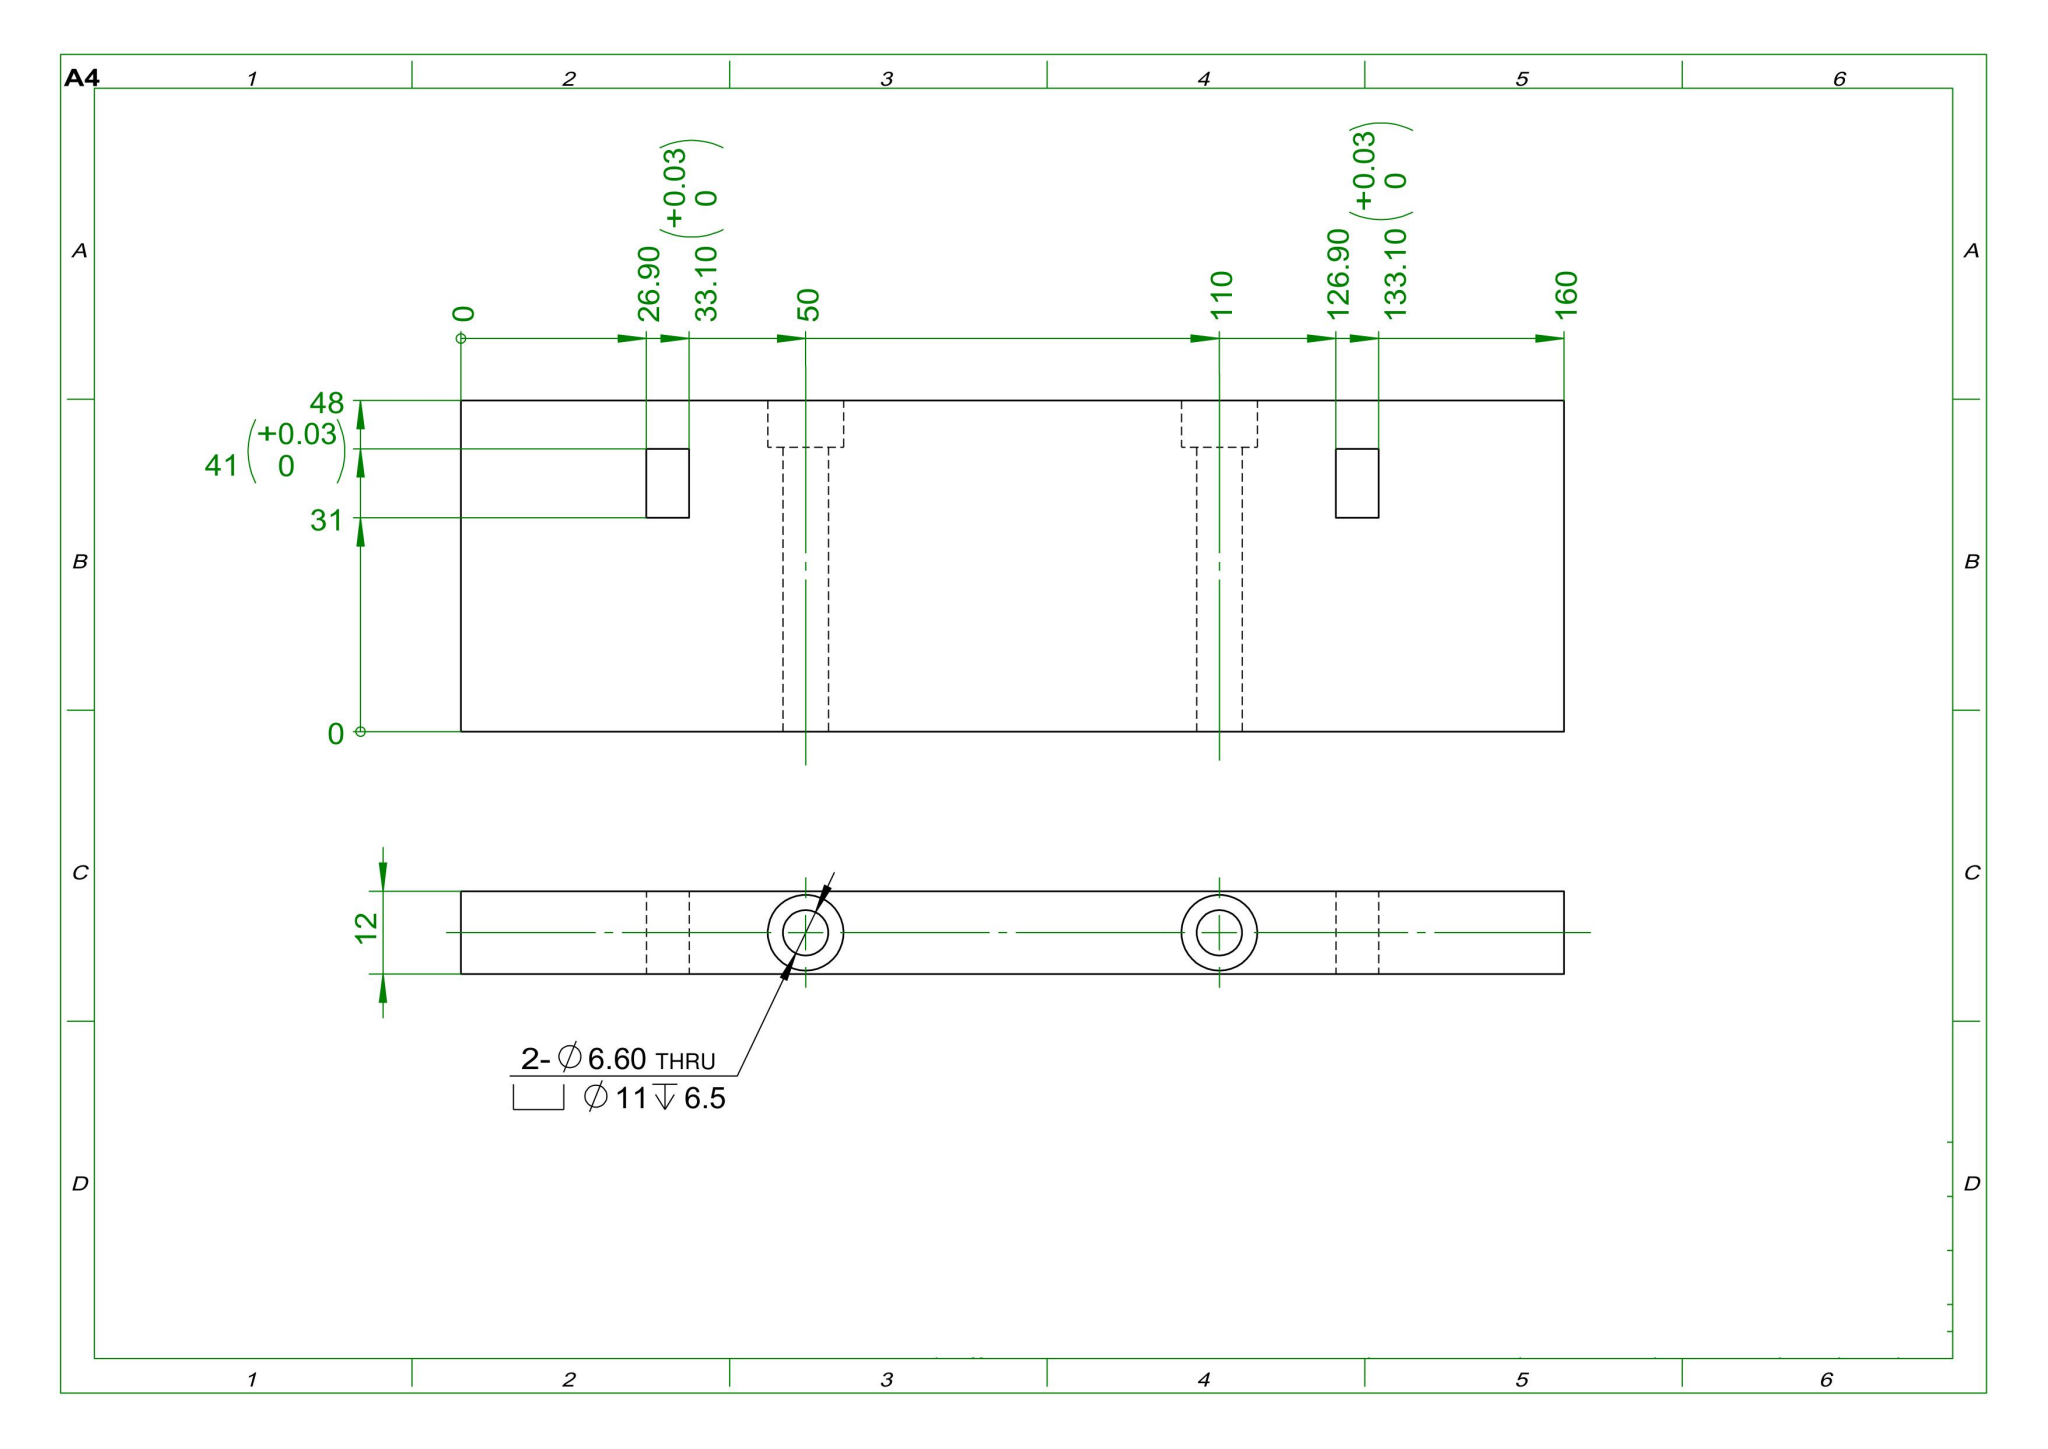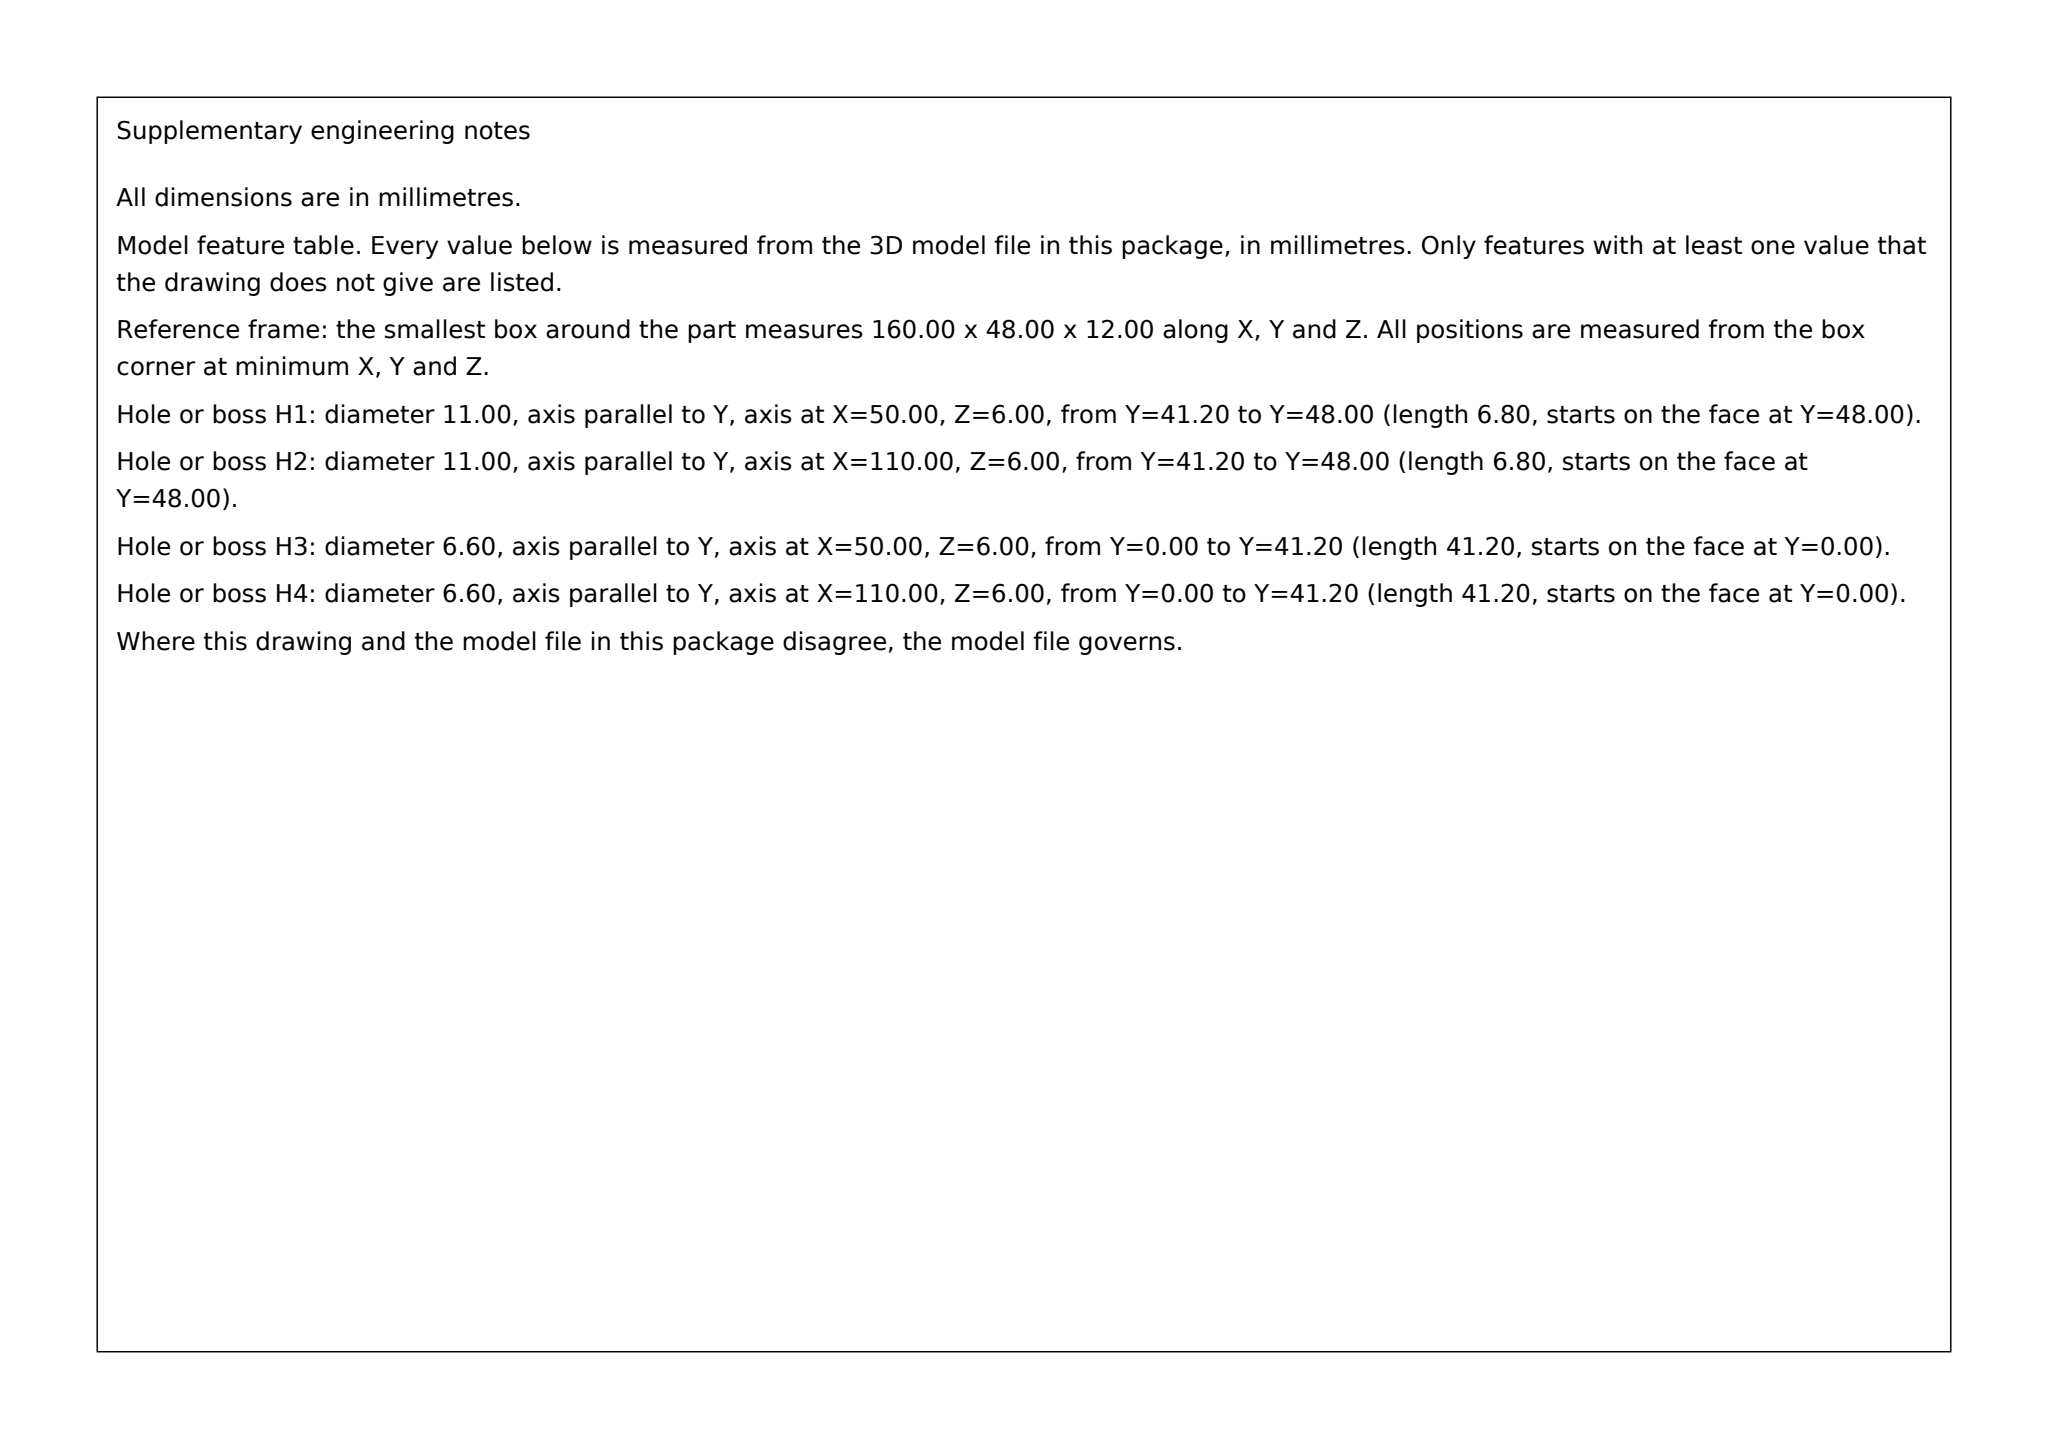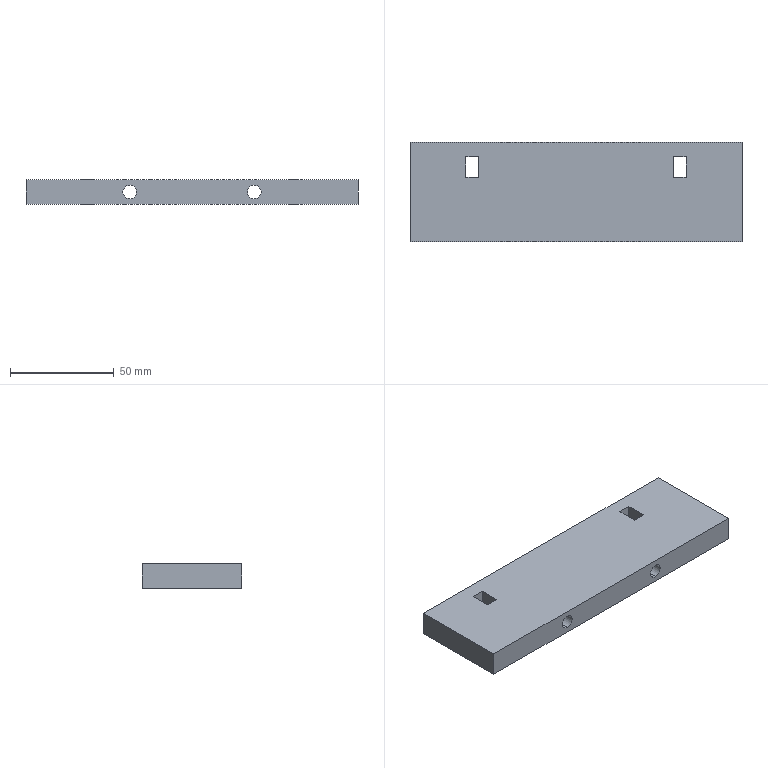Part | SolidWorks | mm | 1 solid | 24 faces | box 160 x 48 x 12 mm | volume 86560 mm3 | plane 16 | cylinder 8 | commonest cylinder face diameters 11 x4 6.6 x4
build123d program:
from build123d import *

# Parameters (mm, degrees)
SKETCH1_W                                            = 160
SKETCH1_H                                            = 48
SKETCH1_W_2                                          = 6.2
SKETCH1_H_2                                          = 10
BOSS_EXTRUDE1_DEPTH                                  = 12
HOLE_SIZE_ACCORDING_TO_HEXAGON_SOCKET_HE_D           = 6.6
HOLE_SIZE_ACCORDING_TO_HEXAGON_SOCKET_HE_CBORE_D     = 11
HOLE_SIZE_ACCORDING_TO_HEXAGON_SOCKET_HE_CBORE_DEPTH = 6.8


with BuildPart() as part:
    # Sketch1 → Boss-Extrude1 (new body)
    with BuildSketch(Plane.XY):
        Rectangle(SKETCH1_W, SKETCH1_H)
        with Locations((50, 12)):
            Rectangle(SKETCH1_W_2, SKETCH1_H_2, mode=Mode.SUBTRACT)
        with Locations((-50, 12)):
            Rectangle(SKETCH1_W_2, SKETCH1_H_2, mode=Mode.SUBTRACT)
    extrude(amount=BOSS_EXTRUDE1_DEPTH)

    # Hole Size_according to_Hexagon Socket He (through all)
    with Locations(Plane(origin=(0, 24, 0), x_dir=(1, 0, 0), z_dir=(0, 1, 0))):
        with Locations((-30, -6), (30, -6)):
            CounterBoreHole(HOLE_SIZE_ACCORDING_TO_HEXAGON_SOCKET_HE_D / 2, HOLE_SIZE_ACCORDING_TO_HEXAGON_SOCKET_HE_CBORE_D / 2, HOLE_SIZE_ACCORDING_TO_HEXAGON_SOCKET_HE_CBORE_DEPTH)


solid = part.part
STEP:
#1=CARTESIAN_POINT('',(-30.,17.2,0.5));
#2=VERTEX_POINT('',#1);
#3=CARTESIAN_POINT('',(-30.,17.2,11.5));
#4=VERTEX_POINT('',#3);
#5=CARTESIAN_POINT('',(-30.,17.2,6.));
#6=DIRECTION('',(0.,1.,0.));
#7=DIRECTION('',(0.,0.,1.));
#8=AXIS2_PLACEMENT_3D('',#5,#6,#7);
#9=CIRCLE('',#8,5.5);
#10=EDGE_CURVE('',#2,#4,#9,.T.);
#11=ORIENTED_EDGE('',*,*,#10,.F.);
#12=CARTESIAN_POINT('',(-30.,24.,0.5));
#13=VERTEX_POINT('',#12);
#14=CARTESIAN_POINT('',(-30.,24.,0.5));
#15=DIRECTION('',(0.,1.,0.));
#16=VECTOR('',#15,1000.);
#17=LINE('',#14,#16);
#18=EDGE_CURVE('',#2,#13,#17,.T.);
#19=ORIENTED_EDGE('',*,*,#18,.T.);
#20=CARTESIAN_POINT('',(-30.,24.,11.5));
#21=VERTEX_POINT('',#20);
#22=CARTESIAN_POINT('',(-30.,24.,6.));
#23=DIRECTION('',(0.,1.,0.));
#24=DIRECTION('',(0.,0.,1.));
#25=AXIS2_PLACEMENT_3D('',#22,#23,#24);
#26=CIRCLE('',#25,5.5);
#27=EDGE_CURVE('',#13,#21,#26,.T.);
#28=ORIENTED_EDGE('',*,*,#27,.T.);
#29=CARTESIAN_POINT('',(-30.,24.,11.5));
#30=DIRECTION('',(0.,1.,0.));
#31=VECTOR('',#30,1000.);
#32=LINE('',#29,#31);
#33=EDGE_CURVE('',#4,#21,#32,.T.);
#34=ORIENTED_EDGE('',*,*,#33,.F.);
#35=EDGE_LOOP('',(#11,#19,#28,#34));
#36=FACE_OUTER_BOUND('',#35,.T.);
#37=CARTESIAN_POINT('',(-30.,24.,6.));
#38=DIRECTION('',(0.,1.,0.));
#39=DIRECTION('',(0.,0.,1.));
#40=AXIS2_PLACEMENT_3D('',#37,#38,#39);
#41=CYLINDRICAL_SURFACE('',#40,5.5);
#42=ADVANCED_FACE('',(#36),#41,.F.);
#43=CARTESIAN_POINT('',(-30.,-24.,2.7));
#44=VERTEX_POINT('',#43);
#45=CARTESIAN_POINT('',(-30.,-24.,9.3));
#46=VERTEX_POINT('',#45);
#47=CARTESIAN_POINT('',(-30.,-24.,6.));
#48=DIRECTION('',(0.,1.,0.));
#49=DIRECTION('',(0.,0.,1.));
#50=AXIS2_PLACEMENT_3D('',#47,#48,#49);
#51=CIRCLE('',#50,3.3);
#52=EDGE_CURVE('',#44,#46,#51,.T.);
#53=ORIENTED_EDGE('',*,*,#52,.F.);
#54=CARTESIAN_POINT('',(-30.,17.2,2.7));
#55=VERTEX_POINT('',#54);
#56=CARTESIAN_POINT('',(-30.,24.,2.7));
#57=DIRECTION('',(0.,1.,0.));
#58=VECTOR('',#57,1000.);
#59=LINE('',#56,#58);
#60=EDGE_CURVE('',#44,#55,#59,.T.);
#61=ORIENTED_EDGE('',*,*,#60,.T.);
#62=CARTESIAN_POINT('',(-30.,17.2,9.3));
#63=VERTEX_POINT('',#62);
#64=CARTESIAN_POINT('',(-30.,17.2,6.));
#65=DIRECTION('',(0.,1.,0.));
#66=DIRECTION('',(0.,0.,1.));
#67=AXIS2_PLACEMENT_3D('',#64,#65,#66);
#68=CIRCLE('',#67,3.3);
#69=EDGE_CURVE('',#55,#63,#68,.T.);
#70=ORIENTED_EDGE('',*,*,#69,.T.);
#71=CARTESIAN_POINT('',(-30.,24.,9.3));
#72=DIRECTION('',(0.,1.,0.));
#73=VECTOR('',#72,1000.);
#74=LINE('',#71,#73);
#75=EDGE_CURVE('',#46,#63,#74,.T.);
#76=ORIENTED_EDGE('',*,*,#75,.F.);
#77=EDGE_LOOP('',(#53,#61,#70,#76));
#78=FACE_OUTER_BOUND('',#77,.T.);
#79=CARTESIAN_POINT('',(-30.,24.,6.));
#80=DIRECTION('',(0.,1.,0.));
#81=DIRECTION('',(0.,0.,1.));
#82=AXIS2_PLACEMENT_3D('',#79,#80,#81);
#83=CYLINDRICAL_SURFACE('',#82,3.3);
#84=ADVANCED_FACE('',(#78),#83,.F.);
#85=CARTESIAN_POINT('',(30.,17.2,0.5));
#86=VERTEX_POINT('',#85);
#87=CARTESIAN_POINT('',(30.,17.2,11.5));
#88=VERTEX_POINT('',#87);
#89=CARTESIAN_POINT('',(30.,17.2,6.));
#90=DIRECTION('',(0.,1.,0.));
#91=DIRECTION('',(0.,0.,1.));
#92=AXIS2_PLACEMENT_3D('',#89,#90,#91);
#93=CIRCLE('',#92,5.5);
#94=EDGE_CURVE('',#86,#88,#93,.T.);
#95=ORIENTED_EDGE('',*,*,#94,.F.);
#96=CARTESIAN_POINT('',(30.,24.,0.5));
#97=VERTEX_POINT('',#96);
#98=CARTESIAN_POINT('',(30.,24.,0.5));
#99=DIRECTION('',(0.,1.,0.));
#100=VECTOR('',#99,1000.);
#101=LINE('',#98,#100);
#102=EDGE_CURVE('',#86,#97,#101,.T.);
#103=ORIENTED_EDGE('',*,*,#102,.T.);
#104=CARTESIAN_POINT('',(30.,24.,11.5));
#105=VERTEX_POINT('',#104);
#106=CARTESIAN_POINT('',(30.,24.,6.));
#107=DIRECTION('',(0.,1.,0.));
#108=DIRECTION('',(0.,0.,1.));
#109=AXIS2_PLACEMENT_3D('',#106,#107,#108);
#110=CIRCLE('',#109,5.5);
#111=EDGE_CURVE('',#97,#105,#110,.T.);
#112=ORIENTED_EDGE('',*,*,#111,.T.);
#113=CARTESIAN_POINT('',(30.,24.,11.5));
#114=DIRECTION('',(0.,1.,0.));
#115=VECTOR('',#114,1000.);
#116=LINE('',#113,#115);
#117=EDGE_CURVE('',#88,#105,#116,.T.);
#118=ORIENTED_EDGE('',*,*,#117,.F.);
#119=EDGE_LOOP('',(#95,#103,#112,#118));
#120=FACE_OUTER_BOUND('',#119,.T.);
#121=CARTESIAN_POINT('',(30.,24.,6.));
#122=DIRECTION('',(0.,1.,0.));
#123=DIRECTION('',(0.,0.,1.));
#124=AXIS2_PLACEMENT_3D('',#121,#122,#123);
#125=CYLINDRICAL_SURFACE('',#124,5.5);
#126=ADVANCED_FACE('',(#120),#125,.F.);
#127=CARTESIAN_POINT('',(30.,-24.,2.7));
#128=VERTEX_POINT('',#127);
#129=CARTESIAN_POINT('',(30.,-24.,9.3));
#130=VERTEX_POINT('',#129);
#131=CARTESIAN_POINT('',(30.,-24.,6.));
#132=DIRECTION('',(0.,1.,0.));
#133=DIRECTION('',(0.,0.,1.));
#134=AXIS2_PLACEMENT_3D('',#131,#132,#133);
#135=CIRCLE('',#134,3.3);
#136=EDGE_CURVE('',#128,#130,#135,.T.);
#137=ORIENTED_EDGE('',*,*,#136,.F.);
#138=CARTESIAN_POINT('',(30.,17.2,2.7));
#139=VERTEX_POINT('',#138);
#140=CARTESIAN_POINT('',(30.,24.,2.7));
#141=DIRECTION('',(0.,1.,0.));
#142=VECTOR('',#141,1000.);
#143=LINE('',#140,#142);
#144=EDGE_CURVE('',#128,#139,#143,.T.);
#145=ORIENTED_EDGE('',*,*,#144,.T.);
#146=CARTESIAN_POINT('',(30.,17.2,9.3));
#147=VERTEX_POINT('',#146);
#148=CARTESIAN_POINT('',(30.,17.2,6.));
#149=DIRECTION('',(0.,1.,0.));
#150=DIRECTION('',(0.,0.,1.));
#151=AXIS2_PLACEMENT_3D('',#148,#149,#150);
#152=CIRCLE('',#151,3.3);
#153=EDGE_CURVE('',#139,#147,#152,.T.);
#154=ORIENTED_EDGE('',*,*,#153,.T.);
#155=CARTESIAN_POINT('',(30.,24.,9.3));
#156=DIRECTION('',(0.,1.,0.));
#157=VECTOR('',#156,1000.);
#158=LINE('',#155,#157);
#159=EDGE_CURVE('',#130,#147,#158,.T.);
#160=ORIENTED_EDGE('',*,*,#159,.F.);
#161=EDGE_LOOP('',(#137,#145,#154,#160));
#162=FACE_OUTER_BOUND('',#161,.T.);
#163=CARTESIAN_POINT('',(30.,24.,6.));
#164=DIRECTION('',(0.,1.,0.));
#165=DIRECTION('',(0.,0.,1.));
#166=AXIS2_PLACEMENT_3D('',#163,#164,#165);
#167=CYLINDRICAL_SURFACE('',#166,3.3);
#168=ADVANCED_FACE('',(#162),#167,.F.);
#169=CARTESIAN_POINT('',(-46.9,7.,12.));
#170=VERTEX_POINT('',#169);
#171=CARTESIAN_POINT('',(-46.9,17.,12.));
#172=VERTEX_POINT('',#171);
#173=CARTESIAN_POINT('',(-46.9,7.,12.));
#174=DIRECTION('',(0.,1.,0.));
#175=VECTOR('',#174,1000.);
#176=LINE('',#173,#175);
#177=EDGE_CURVE('',#170,#172,#176,.T.);
#178=ORIENTED_EDGE('',*,*,#177,.F.);
#179=CARTESIAN_POINT('',(-53.1,7.,12.));
#180=VERTEX_POINT('',#179);
#181=CARTESIAN_POINT('',(-53.1,7.,12.));
#182=DIRECTION('',(1.,0.,0.));
#183=VECTOR('',#182,1000.);
#184=LINE('',#181,#183);
#185=EDGE_CURVE('',#180,#170,#184,.T.);
#186=ORIENTED_EDGE('',*,*,#185,.F.);
#187=CARTESIAN_POINT('',(-53.1,17.,12.));
#188=VERTEX_POINT('',#187);
#189=CARTESIAN_POINT('',(-53.1,7.,12.));
#190=DIRECTION('',(0.,-1.,0.));
#191=VECTOR('',#190,1000.);
#192=LINE('',#189,#191);
#193=EDGE_CURVE('',#188,#180,#192,.T.);
#194=ORIENTED_EDGE('',*,*,#193,.F.);
#195=CARTESIAN_POINT('',(-53.1,17.,12.));
#196=DIRECTION('',(-1.,0.,0.));
#197=VECTOR('',#196,1000.);
#198=LINE('',#195,#197);
#199=EDGE_CURVE('',#172,#188,#198,.T.);
#200=ORIENTED_EDGE('',*,*,#199,.F.);
#201=EDGE_LOOP('',(#178,#186,#194,#200));
#202=FACE_BOUND('',#201,.T.);
#203=CARTESIAN_POINT('',(80.,-24.,12.));
#204=VERTEX_POINT('',#203);
#205=CARTESIAN_POINT('',(80.,24.,12.));
#206=VERTEX_POINT('',#205);
#207=CARTESIAN_POINT('',(80.,-24.,12.));
#208=DIRECTION('',(0.,1.,0.));
#209=VECTOR('',#208,1000.);
#210=LINE('',#207,#209);
#211=EDGE_CURVE('',#204,#206,#210,.T.);
#212=ORIENTED_EDGE('',*,*,#211,.T.);
#213=CARTESIAN_POINT('',(-80.,24.,12.));
#214=VERTEX_POINT('',#213);
#215=CARTESIAN_POINT('',(-80.,24.,12.));
#216=DIRECTION('',(-1.,0.,0.));
#217=VECTOR('',#216,1000.);
#218=LINE('',#215,#217);
#219=EDGE_CURVE('',#206,#214,#218,.T.);
#220=ORIENTED_EDGE('',*,*,#219,.T.);
#221=CARTESIAN_POINT('',(-80.,-24.,12.));
#222=VERTEX_POINT('',#221);
#223=CARTESIAN_POINT('',(-80.,-24.,12.));
#224=DIRECTION('',(0.,-1.,0.));
#225=VECTOR('',#224,1000.);
#226=LINE('',#223,#225);
#227=EDGE_CURVE('',#214,#222,#226,.T.);
#228=ORIENTED_EDGE('',*,*,#227,.T.);
#229=CARTESIAN_POINT('',(-80.,-24.,12.));
#230=DIRECTION('',(1.,0.,0.));
#231=VECTOR('',#230,1000.);
#232=LINE('',#229,#231);
#233=EDGE_CURVE('',#222,#204,#232,.T.);
#234=ORIENTED_EDGE('',*,*,#233,.T.);
#235=EDGE_LOOP('',(#212,#220,#228,#234));
#236=FACE_OUTER_BOUND('',#235,.T.);
#237=CARTESIAN_POINT('',(53.1,7.,12.));
#238=VERTEX_POINT('',#237);
#239=CARTESIAN_POINT('',(53.1,17.,12.));
#240=VERTEX_POINT('',#239);
#241=CARTESIAN_POINT('',(53.1,7.,12.));
#242=DIRECTION('',(0.,1.,0.));
#243=VECTOR('',#242,1000.);
#244=LINE('',#241,#243);
#245=EDGE_CURVE('',#238,#240,#244,.T.);
#246=ORIENTED_EDGE('',*,*,#245,.F.);
#247=CARTESIAN_POINT('',(46.9,7.,12.));
#248=VERTEX_POINT('',#247);
#249=CARTESIAN_POINT('',(53.1,7.,12.));
#250=DIRECTION('',(1.,0.,0.));
#251=VECTOR('',#250,1000.);
#252=LINE('',#249,#251);
#253=EDGE_CURVE('',#248,#238,#252,.T.);
#254=ORIENTED_EDGE('',*,*,#253,.F.);
#255=CARTESIAN_POINT('',(46.9,17.,12.));
#256=VERTEX_POINT('',#255);
#257=CARTESIAN_POINT('',(46.9,7.,12.));
#258=DIRECTION('',(0.,-1.,0.));
#259=VECTOR('',#258,1000.);
#260=LINE('',#257,#259);
#261=EDGE_CURVE('',#256,#248,#260,.T.);
#262=ORIENTED_EDGE('',*,*,#261,.F.);
#263=CARTESIAN_POINT('',(53.1,17.,12.));
#264=DIRECTION('',(-1.,0.,0.));
#265=VECTOR('',#264,1000.);
#266=LINE('',#263,#265);
#267=EDGE_CURVE('',#240,#256,#266,.T.);
#268=ORIENTED_EDGE('',*,*,#267,.F.);
#269=EDGE_LOOP('',(#246,#254,#262,#268));
#270=FACE_BOUND('',#269,.T.);
#271=CARTESIAN_POINT('',(0.,0.,12.));
#272=DIRECTION('',(0.,0.,-1.));
#273=DIRECTION('',(-1.,0.,0.));
#274=AXIS2_PLACEMENT_3D('',#271,#272,#273);
#275=PLANE('',#274);
#276=ADVANCED_FACE('',(#202,#236,#270),#275,.F.);
#277=CARTESIAN_POINT('',(-53.1,7.,0.));
#278=VERTEX_POINT('',#277);
#279=CARTESIAN_POINT('',(-46.9,7.,0.));
#280=VERTEX_POINT('',#279);
#281=CARTESIAN_POINT('',(-53.1,7.,0.));
#282=DIRECTION('',(1.,0.,0.));
#283=VECTOR('',#282,1000.);
#284=LINE('',#281,#283);
#285=EDGE_CURVE('',#278,#280,#284,.T.);
#286=ORIENTED_EDGE('',*,*,#285,.T.);
#287=CARTESIAN_POINT('',(-46.9,17.,0.));
#288=VERTEX_POINT('',#287);
#289=CARTESIAN_POINT('',(-46.9,7.,0.));
#290=DIRECTION('',(0.,1.,0.));
#291=VECTOR('',#290,1000.);
#292=LINE('',#289,#291);
#293=EDGE_CURVE('',#280,#288,#292,.T.);
#294=ORIENTED_EDGE('',*,*,#293,.T.);
#295=CARTESIAN_POINT('',(-53.1,17.,0.));
#296=VERTEX_POINT('',#295);
#297=CARTESIAN_POINT('',(-53.1,17.,0.));
#298=DIRECTION('',(-1.,0.,0.));
#299=VECTOR('',#298,1000.);
#300=LINE('',#297,#299);
#301=EDGE_CURVE('',#288,#296,#300,.T.);
#302=ORIENTED_EDGE('',*,*,#301,.T.);
#303=CARTESIAN_POINT('',(-53.1,7.,0.));
#304=DIRECTION('',(0.,-1.,0.));
#305=VECTOR('',#304,1000.);
#306=LINE('',#303,#305);
#307=EDGE_CURVE('',#296,#278,#306,.T.);
#308=ORIENTED_EDGE('',*,*,#307,.T.);
#309=EDGE_LOOP('',(#286,#294,#302,#308));
#310=FACE_BOUND('',#309,.T.);
#311=CARTESIAN_POINT('',(80.,-24.,0.));
#312=VERTEX_POINT('',#311);
#313=CARTESIAN_POINT('',(80.,24.,0.));
#314=VERTEX_POINT('',#313);
#315=CARTESIAN_POINT('',(80.,-24.,0.));
#316=DIRECTION('',(0.,1.,0.));
#317=VECTOR('',#316,1000.);
#318=LINE('',#315,#317);
#319=EDGE_CURVE('',#312,#314,#318,.T.);
#320=ORIENTED_EDGE('',*,*,#319,.F.);
#321=CARTESIAN_POINT('',(-80.,-24.,0.));
#322=VERTEX_POINT('',#321);
#323=CARTESIAN_POINT('',(-80.,-24.,0.));
#324=DIRECTION('',(1.,0.,0.));
#325=VECTOR('',#324,1000.);
#326=LINE('',#323,#325);
#327=EDGE_CURVE('',#322,#312,#326,.T.);
#328=ORIENTED_EDGE('',*,*,#327,.F.);
#329=CARTESIAN_POINT('',(-80.,24.,0.));
#330=VERTEX_POINT('',#329);
#331=CARTESIAN_POINT('',(-80.,-24.,0.));
#332=DIRECTION('',(0.,-1.,0.));
#333=VECTOR('',#332,1000.);
#334=LINE('',#331,#333);
#335=EDGE_CURVE('',#330,#322,#334,.T.);
#336=ORIENTED_EDGE('',*,*,#335,.F.);
#337=CARTESIAN_POINT('',(-80.,24.,0.));
#338=DIRECTION('',(-1.,0.,0.));
#339=VECTOR('',#338,1000.);
#340=LINE('',#337,#339);
#341=EDGE_CURVE('',#314,#330,#340,.T.);
#342=ORIENTED_EDGE('',*,*,#341,.F.);
#343=EDGE_LOOP('',(#320,#328,#336,#342));
#344=FACE_OUTER_BOUND('',#343,.T.);
#345=CARTESIAN_POINT('',(46.9,7.,0.));
#346=VERTEX_POINT('',#345);
#347=CARTESIAN_POINT('',(53.1,7.,0.));
#348=VERTEX_POINT('',#347);
#349=CARTESIAN_POINT('',(53.1,7.,0.));
#350=DIRECTION('',(1.,0.,0.));
#351=VECTOR('',#350,1000.);
#352=LINE('',#349,#351);
#353=EDGE_CURVE('',#346,#348,#352,.T.);
#354=ORIENTED_EDGE('',*,*,#353,.T.);
#355=CARTESIAN_POINT('',(53.1,17.,0.));
#356=VERTEX_POINT('',#355);
#357=CARTESIAN_POINT('',(53.1,7.,0.));
#358=DIRECTION('',(0.,1.,0.));
#359=VECTOR('',#358,1000.);
#360=LINE('',#357,#359);
#361=EDGE_CURVE('',#348,#356,#360,.T.);
#362=ORIENTED_EDGE('',*,*,#361,.T.);
#363=CARTESIAN_POINT('',(46.9,17.,0.));
#364=VERTEX_POINT('',#363);
#365=CARTESIAN_POINT('',(53.1,17.,0.));
#366=DIRECTION('',(-1.,0.,0.));
#367=VECTOR('',#366,1000.);
#368=LINE('',#365,#367);
#369=EDGE_CURVE('',#356,#364,#368,.T.);
#370=ORIENTED_EDGE('',*,*,#369,.T.);
#371=CARTESIAN_POINT('',(46.9,7.,0.));
#372=DIRECTION('',(0.,-1.,0.));
#373=VECTOR('',#372,1000.);
#374=LINE('',#371,#373);
#375=EDGE_CURVE('',#364,#346,#374,.T.);
#376=ORIENTED_EDGE('',*,*,#375,.T.);
#377=EDGE_LOOP('',(#354,#362,#370,#376));
#378=FACE_BOUND('',#377,.T.);
#379=CARTESIAN_POINT('',(0.,0.,0.));
#380=DIRECTION('',(0.,0.,-1.));
#381=DIRECTION('',(-1.,0.,0.));
#382=AXIS2_PLACEMENT_3D('',#379,#380,#381);
#383=PLANE('',#382);
#384=ADVANCED_FACE('',(#310,#344,#378),#383,.T.);
#385=ORIENTED_EDGE('',*,*,#319,.T.);
#386=CARTESIAN_POINT('',(80.,24.,12.));
#387=DIRECTION('',(0.,0.,-1.));
#388=VECTOR('',#387,1000.);
#389=LINE('',#386,#388);
#390=EDGE_CURVE('',#206,#314,#389,.T.);
#391=ORIENTED_EDGE('',*,*,#390,.F.);
#392=ORIENTED_EDGE('',*,*,#211,.F.);
#393=CARTESIAN_POINT('',(80.,-24.,12.));
#394=DIRECTION('',(0.,0.,-1.));
#395=VECTOR('',#394,1000.);
#396=LINE('',#393,#395);
#397=EDGE_CURVE('',#204,#312,#396,.T.);
#398=ORIENTED_EDGE('',*,*,#397,.T.);
#399=EDGE_LOOP('',(#385,#391,#392,#398));
#400=FACE_OUTER_BOUND('',#399,.T.);
#401=CARTESIAN_POINT('',(80.,-24.,12.));
#402=DIRECTION('',(-1.,0.,0.));
#403=DIRECTION('',(0.,0.,1.));
#404=AXIS2_PLACEMENT_3D('',#401,#402,#403);
#405=PLANE('',#404);
#406=ADVANCED_FACE('',(#400),#405,.F.);
#407=CARTESIAN_POINT('',(-30.,24.,6.));
#408=DIRECTION('',(0.,1.,0.));
#409=DIRECTION('',(0.,0.,1.));
#410=AXIS2_PLACEMENT_3D('',#407,#408,#409);
#411=CIRCLE('',#410,5.5);
#412=EDGE_CURVE('',#21,#13,#411,.T.);
#413=ORIENTED_EDGE('',*,*,#412,.F.);
#414=ORIENTED_EDGE('',*,*,#27,.F.);
#415=EDGE_LOOP('',(#413,#414));
#416=FACE_BOUND('',#415,.T.);
#417=CARTESIAN_POINT('',(30.,24.,6.));
#418=DIRECTION('',(0.,1.,0.));
#419=DIRECTION('',(0.,0.,1.));
#420=AXIS2_PLACEMENT_3D('',#417,#418,#419);
#421=CIRCLE('',#420,5.5);
#422=EDGE_CURVE('',#105,#97,#421,.T.);
#423=ORIENTED_EDGE('',*,*,#422,.F.);
#424=ORIENTED_EDGE('',*,*,#111,.F.);
#425=EDGE_LOOP('',(#423,#424));
#426=FACE_BOUND('',#425,.T.);
#427=ORIENTED_EDGE('',*,*,#341,.T.);
#428=CARTESIAN_POINT('',(-80.,24.,12.));
#429=DIRECTION('',(0.,0.,-1.));
#430=VECTOR('',#429,1000.);
#431=LINE('',#428,#430);
#432=EDGE_CURVE('',#214,#330,#431,.T.);
#433=ORIENTED_EDGE('',*,*,#432,.F.);
#434=ORIENTED_EDGE('',*,*,#219,.F.);
#435=ORIENTED_EDGE('',*,*,#390,.T.);
#436=EDGE_LOOP('',(#427,#433,#434,#435));
#437=FACE_OUTER_BOUND('',#436,.T.);
#438=CARTESIAN_POINT('',(-80.,24.,12.));
#439=DIRECTION('',(0.,-1.,0.));
#440=DIRECTION('',(0.,0.,-1.));
#441=AXIS2_PLACEMENT_3D('',#438,#439,#440);
#442=PLANE('',#441);
#443=ADVANCED_FACE('',(#416,#426,#437),#442,.F.);
#444=ORIENTED_EDGE('',*,*,#335,.T.);
#445=CARTESIAN_POINT('',(-80.,-24.,12.));
#446=DIRECTION('',(0.,0.,-1.));
#447=VECTOR('',#446,1000.);
#448=LINE('',#445,#447);
#449=EDGE_CURVE('',#222,#322,#448,.T.);
#450=ORIENTED_EDGE('',*,*,#449,.F.);
#451=ORIENTED_EDGE('',*,*,#227,.F.);
#452=ORIENTED_EDGE('',*,*,#432,.T.);
#453=EDGE_LOOP('',(#444,#450,#451,#452));
#454=FACE_OUTER_BOUND('',#453,.T.);
#455=CARTESIAN_POINT('',(-80.,-24.,12.));
#456=DIRECTION('',(1.,0.,0.));
#457=DIRECTION('',(0.,0.,-1.));
#458=AXIS2_PLACEMENT_3D('',#455,#456,#457);
#459=PLANE('',#458);
#460=ADVANCED_FACE('',(#454),#459,.F.);
#461=CARTESIAN_POINT('',(-30.,-24.,6.));
#462=DIRECTION('',(0.,1.,0.));
#463=DIRECTION('',(0.,0.,1.));
#464=AXIS2_PLACEMENT_3D('',#461,#462,#463);
#465=CIRCLE('',#464,3.3);
#466=EDGE_CURVE('',#46,#44,#465,.T.);
#467=ORIENTED_EDGE('',*,*,#466,.T.);
#468=ORIENTED_EDGE('',*,*,#52,.T.);
#469=EDGE_LOOP('',(#467,#468));
#470=FACE_BOUND('',#469,.T.);
#471=CARTESIAN_POINT('',(30.,-24.,6.));
#472=DIRECTION('',(0.,1.,0.));
#473=DIRECTION('',(0.,0.,1.));
#474=AXIS2_PLACEMENT_3D('',#471,#472,#473);
#475=CIRCLE('',#474,3.3);
#476=EDGE_CURVE('',#130,#128,#475,.T.);
#477=ORIENTED_EDGE('',*,*,#476,.T.);
#478=ORIENTED_EDGE('',*,*,#136,.T.);
#479=EDGE_LOOP('',(#477,#478));
#480=FACE_BOUND('',#479,.T.);
#481=ORIENTED_EDGE('',*,*,#327,.T.);
#482=ORIENTED_EDGE('',*,*,#397,.F.);
#483=ORIENTED_EDGE('',*,*,#233,.F.);
#484=ORIENTED_EDGE('',*,*,#449,.T.);
#485=EDGE_LOOP('',(#481,#482,#483,#484));
#486=FACE_OUTER_BOUND('',#485,.T.);
#487=CARTESIAN_POINT('',(-80.,-24.,12.));
#488=DIRECTION('',(0.,1.,0.));
#489=DIRECTION('',(0.,0.,1.));
#490=AXIS2_PLACEMENT_3D('',#487,#488,#489);
#491=PLANE('',#490);
#492=ADVANCED_FACE('',(#470,#480,#486),#491,.F.);
#493=ORIENTED_EDGE('',*,*,#293,.F.);
#494=CARTESIAN_POINT('',(-46.9,7.,12.));
#495=DIRECTION('',(0.,0.,-1.));
#496=VECTOR('',#495,1000.);
#497=LINE('',#494,#496);
#498=EDGE_CURVE('',#170,#280,#497,.T.);
#499=ORIENTED_EDGE('',*,*,#498,.F.);
#500=ORIENTED_EDGE('',*,*,#177,.T.);
#501=CARTESIAN_POINT('',(-46.9,17.,12.));
#502=DIRECTION('',(0.,0.,-1.));
#503=VECTOR('',#502,1000.);
#504=LINE('',#501,#503);
#505=EDGE_CURVE('',#172,#288,#504,.T.);
#506=ORIENTED_EDGE('',*,*,#505,.T.);
#507=EDGE_LOOP('',(#493,#499,#500,#506));
#508=FACE_OUTER_BOUND('',#507,.T.);
#509=CARTESIAN_POINT('',(-46.9,7.,12.));
#510=DIRECTION('',(-1.,0.,0.));
#511=DIRECTION('',(0.,0.,1.));
#512=AXIS2_PLACEMENT_3D('',#509,#510,#511);
#513=PLANE('',#512);
#514=ADVANCED_FACE('',(#508),#513,.T.);
#515=ORIENTED_EDGE('',*,*,#301,.F.);
#516=ORIENTED_EDGE('',*,*,#505,.F.);
#517=ORIENTED_EDGE('',*,*,#199,.T.);
#518=CARTESIAN_POINT('',(-53.1,17.,12.));
#519=DIRECTION('',(0.,0.,-1.));
#520=VECTOR('',#519,1000.);
#521=LINE('',#518,#520);
#522=EDGE_CURVE('',#188,#296,#521,.T.);
#523=ORIENTED_EDGE('',*,*,#522,.T.);
#524=EDGE_LOOP('',(#515,#516,#517,#523));
#525=FACE_OUTER_BOUND('',#524,.T.);
#526=CARTESIAN_POINT('',(-53.1,17.,12.));
#527=DIRECTION('',(0.,-1.,0.));
#528=DIRECTION('',(0.,0.,-1.));
#529=AXIS2_PLACEMENT_3D('',#526,#527,#528);
#530=PLANE('',#529);
#531=ADVANCED_FACE('',(#525),#530,.T.);
#532=ORIENTED_EDGE('',*,*,#307,.F.);
#533=ORIENTED_EDGE('',*,*,#522,.F.);
#534=ORIENTED_EDGE('',*,*,#193,.T.);
#535=CARTESIAN_POINT('',(-53.1,7.,12.));
#536=DIRECTION('',(0.,0.,-1.));
#537=VECTOR('',#536,1000.);
#538=LINE('',#535,#537);
#539=EDGE_CURVE('',#180,#278,#538,.T.);
#540=ORIENTED_EDGE('',*,*,#539,.T.);
#541=EDGE_LOOP('',(#532,#533,#534,#540));
#542=FACE_OUTER_BOUND('',#541,.T.);
#543=CARTESIAN_POINT('',(-53.1,7.,12.));
#544=DIRECTION('',(1.,0.,0.));
#545=DIRECTION('',(0.,0.,-1.));
#546=AXIS2_PLACEMENT_3D('',#543,#544,#545);
#547=PLANE('',#546);
#548=ADVANCED_FACE('',(#542),#547,.T.);
#549=ORIENTED_EDGE('',*,*,#285,.F.);
#550=ORIENTED_EDGE('',*,*,#539,.F.);
#551=ORIENTED_EDGE('',*,*,#185,.T.);
#552=ORIENTED_EDGE('',*,*,#498,.T.);
#553=EDGE_LOOP('',(#549,#550,#551,#552));
#554=FACE_OUTER_BOUND('',#553,.T.);
#555=CARTESIAN_POINT('',(-53.1,7.,12.));
#556=DIRECTION('',(0.,1.,0.));
#557=DIRECTION('',(0.,0.,1.));
#558=AXIS2_PLACEMENT_3D('',#555,#556,#557);
#559=PLANE('',#558);
#560=ADVANCED_FACE('',(#554),#559,.T.);
#561=ORIENTED_EDGE('',*,*,#361,.F.);
#562=CARTESIAN_POINT('',(53.1,7.,12.));
#563=DIRECTION('',(0.,0.,-1.));
#564=VECTOR('',#563,1000.);
#565=LINE('',#562,#564);
#566=EDGE_CURVE('',#238,#348,#565,.T.);
#567=ORIENTED_EDGE('',*,*,#566,.F.);
#568=ORIENTED_EDGE('',*,*,#245,.T.);
#569=CARTESIAN_POINT('',(53.1,17.,12.));
#570=DIRECTION('',(0.,0.,-1.));
#571=VECTOR('',#570,1000.);
#572=LINE('',#569,#571);
#573=EDGE_CURVE('',#240,#356,#572,.T.);
#574=ORIENTED_EDGE('',*,*,#573,.T.);
#575=EDGE_LOOP('',(#561,#567,#568,#574));
#576=FACE_OUTER_BOUND('',#575,.T.);
#577=CARTESIAN_POINT('',(53.1,7.,12.));
#578=DIRECTION('',(-1.,0.,0.));
#579=DIRECTION('',(0.,0.,1.));
#580=AXIS2_PLACEMENT_3D('',#577,#578,#579);
#581=PLANE('',#580);
#582=ADVANCED_FACE('',(#576),#581,.T.);
#583=ORIENTED_EDGE('',*,*,#369,.F.);
#584=ORIENTED_EDGE('',*,*,#573,.F.);
#585=ORIENTED_EDGE('',*,*,#267,.T.);
#586=CARTESIAN_POINT('',(46.9,17.,12.));
#587=DIRECTION('',(0.,0.,-1.));
#588=VECTOR('',#587,1000.);
#589=LINE('',#586,#588);
#590=EDGE_CURVE('',#256,#364,#589,.T.);
#591=ORIENTED_EDGE('',*,*,#590,.T.);
#592=EDGE_LOOP('',(#583,#584,#585,#591));
#593=FACE_OUTER_BOUND('',#592,.T.);
#594=CARTESIAN_POINT('',(53.1,17.,12.));
#595=DIRECTION('',(0.,-1.,0.));
#596=DIRECTION('',(0.,0.,-1.));
#597=AXIS2_PLACEMENT_3D('',#594,#595,#596);
#598=PLANE('',#597);
#599=ADVANCED_FACE('',(#593),#598,.T.);
#600=ORIENTED_EDGE('',*,*,#375,.F.);
#601=ORIENTED_EDGE('',*,*,#590,.F.);
#602=ORIENTED_EDGE('',*,*,#261,.T.);
#603=CARTESIAN_POINT('',(46.9,7.,12.));
#604=DIRECTION('',(0.,0.,-1.));
#605=VECTOR('',#604,1000.);
#606=LINE('',#603,#605);
#607=EDGE_CURVE('',#248,#346,#606,.T.);
#608=ORIENTED_EDGE('',*,*,#607,.T.);
#609=EDGE_LOOP('',(#600,#601,#602,#608));
#610=FACE_OUTER_BOUND('',#609,.T.);
#611=CARTESIAN_POINT('',(46.9,7.,12.));
#612=DIRECTION('',(1.,0.,0.));
#613=DIRECTION('',(0.,0.,-1.));
#614=AXIS2_PLACEMENT_3D('',#611,#612,#613);
#615=PLANE('',#614);
#616=ADVANCED_FACE('',(#610),#615,.T.);
#617=ORIENTED_EDGE('',*,*,#353,.F.);
#618=ORIENTED_EDGE('',*,*,#607,.F.);
#619=ORIENTED_EDGE('',*,*,#253,.T.);
#620=ORIENTED_EDGE('',*,*,#566,.T.);
#621=EDGE_LOOP('',(#617,#618,#619,#620));
#622=FACE_OUTER_BOUND('',#621,.T.);
#623=CARTESIAN_POINT('',(53.1,7.,12.));
#624=DIRECTION('',(0.,1.,0.));
#625=DIRECTION('',(0.,0.,1.));
#626=AXIS2_PLACEMENT_3D('',#623,#624,#625);
#627=PLANE('',#626);
#628=ADVANCED_FACE('',(#622),#627,.T.);
#629=ORIENTED_EDGE('',*,*,#144,.F.);
#630=ORIENTED_EDGE('',*,*,#476,.F.);
#631=ORIENTED_EDGE('',*,*,#159,.T.);
#632=CARTESIAN_POINT('',(30.,17.2,6.));
#633=DIRECTION('',(0.,1.,0.));
#634=DIRECTION('',(0.,0.,1.));
#635=AXIS2_PLACEMENT_3D('',#632,#633,#634);
#636=CIRCLE('',#635,3.3);
#637=EDGE_CURVE('',#147,#139,#636,.T.);
#638=ORIENTED_EDGE('',*,*,#637,.T.);
#639=EDGE_LOOP('',(#629,#630,#631,#638));
#640=FACE_OUTER_BOUND('',#639,.T.);
#641=CARTESIAN_POINT('',(30.,24.,6.));
#642=DIRECTION('',(0.,1.,0.));
#643=DIRECTION('',(0.,0.,1.));
#644=AXIS2_PLACEMENT_3D('',#641,#642,#643);
#645=CYLINDRICAL_SURFACE('',#644,3.3);
#646=ADVANCED_FACE('',(#640),#645,.F.);
#647=ORIENTED_EDGE('',*,*,#637,.F.);
#648=ORIENTED_EDGE('',*,*,#153,.F.);
#649=EDGE_LOOP('',(#647,#648));
#650=FACE_BOUND('',#649,.T.);
#651=CARTESIAN_POINT('',(30.,17.2,6.));
#652=DIRECTION('',(0.,1.,0.));
#653=DIRECTION('',(0.,0.,1.));
#654=AXIS2_PLACEMENT_3D('',#651,#652,#653);
#655=CIRCLE('',#654,5.5);
#656=EDGE_CURVE('',#88,#86,#655,.T.);
#657=ORIENTED_EDGE('',*,*,#656,.T.);
#658=ORIENTED_EDGE('',*,*,#94,.T.);
#659=EDGE_LOOP('',(#657,#658));
#660=FACE_OUTER_BOUND('',#659,.T.);
#661=CARTESIAN_POINT('',(33.3,17.2,6.));
#662=DIRECTION('',(0.,-1.,0.));
#663=DIRECTION('',(0.,0.,-1.));
#664=AXIS2_PLACEMENT_3D('',#661,#662,#663);
#665=PLANE('',#664);
#666=ADVANCED_FACE('',(#650,#660),#665,.F.);
#667=ORIENTED_EDGE('',*,*,#102,.F.);
#668=ORIENTED_EDGE('',*,*,#656,.F.);
#669=ORIENTED_EDGE('',*,*,#117,.T.);
#670=ORIENTED_EDGE('',*,*,#422,.T.);
#671=EDGE_LOOP('',(#667,#668,#669,#670));
#672=FACE_OUTER_BOUND('',#671,.T.);
#673=CARTESIAN_POINT('',(30.,24.,6.));
#674=DIRECTION('',(0.,1.,0.));
#675=DIRECTION('',(0.,0.,1.));
#676=AXIS2_PLACEMENT_3D('',#673,#674,#675);
#677=CYLINDRICAL_SURFACE('',#676,5.5);
#678=ADVANCED_FACE('',(#672),#677,.F.);
#679=ORIENTED_EDGE('',*,*,#60,.F.);
#680=ORIENTED_EDGE('',*,*,#466,.F.);
#681=ORIENTED_EDGE('',*,*,#75,.T.);
#682=CARTESIAN_POINT('',(-30.,17.2,6.));
#683=DIRECTION('',(0.,1.,0.));
#684=DIRECTION('',(0.,0.,1.));
#685=AXIS2_PLACEMENT_3D('',#682,#683,#684);
#686=CIRCLE('',#685,3.3);
#687=EDGE_CURVE('',#63,#55,#686,.T.);
#688=ORIENTED_EDGE('',*,*,#687,.T.);
#689=EDGE_LOOP('',(#679,#680,#681,#688));
#690=FACE_OUTER_BOUND('',#689,.T.);
#691=CARTESIAN_POINT('',(-30.,24.,6.));
#692=DIRECTION('',(0.,1.,0.));
#693=DIRECTION('',(0.,0.,1.));
#694=AXIS2_PLACEMENT_3D('',#691,#692,#693);
#695=CYLINDRICAL_SURFACE('',#694,3.3);
#696=ADVANCED_FACE('',(#690),#695,.F.);
#697=ORIENTED_EDGE('',*,*,#687,.F.);
#698=ORIENTED_EDGE('',*,*,#69,.F.);
#699=EDGE_LOOP('',(#697,#698));
#700=FACE_BOUND('',#699,.T.);
#701=CARTESIAN_POINT('',(-30.,17.2,6.));
#702=DIRECTION('',(0.,1.,0.));
#703=DIRECTION('',(0.,0.,1.));
#704=AXIS2_PLACEMENT_3D('',#701,#702,#703);
#705=CIRCLE('',#704,5.5);
#706=EDGE_CURVE('',#4,#2,#705,.T.);
#707=ORIENTED_EDGE('',*,*,#706,.T.);
#708=ORIENTED_EDGE('',*,*,#10,.T.);
#709=EDGE_LOOP('',(#707,#708));
#710=FACE_OUTER_BOUND('',#709,.T.);
#711=CARTESIAN_POINT('',(-26.7,17.2,6.));
#712=DIRECTION('',(0.,-1.,0.));
#713=DIRECTION('',(0.,0.,-1.));
#714=AXIS2_PLACEMENT_3D('',#711,#712,#713);
#715=PLANE('',#714);
#716=ADVANCED_FACE('',(#700,#710),#715,.F.);
#717=ORIENTED_EDGE('',*,*,#18,.F.);
#718=ORIENTED_EDGE('',*,*,#706,.F.);
#719=ORIENTED_EDGE('',*,*,#33,.T.);
#720=ORIENTED_EDGE('',*,*,#412,.T.);
#721=EDGE_LOOP('',(#717,#718,#719,#720));
#722=FACE_OUTER_BOUND('',#721,.T.);
#723=CARTESIAN_POINT('',(-30.,24.,6.));
#724=DIRECTION('',(0.,1.,0.));
#725=DIRECTION('',(0.,0.,1.));
#726=AXIS2_PLACEMENT_3D('',#723,#724,#725);
#727=CYLINDRICAL_SURFACE('',#726,5.5);
#728=ADVANCED_FACE('',(#722),#727,.F.);
#729=CLOSED_SHELL('',(#42,#84,#126,#168,#276,#384,#406,#443,#460,#492,#514,#531,#548,#560,#582,#599,#616,#628,#646,#666,#678,#696,#716,#728));
#730=MANIFOLD_SOLID_BREP('',#729);
#731=CARTESIAN_POINT('',(0.,0.,0.));
#732=DIRECTION('',(0.,0.,1.));
#733=DIRECTION('',(1.,0.,0.));
#734=AXIS2_PLACEMENT_3D('',#731,#732,#733);
#735=(LENGTH_UNIT()NAMED_UNIT(*)SI_UNIT(.MILLI.,.METRE.));
#736=UNCERTAINTY_MEASURE_WITH_UNIT(LENGTH_MEASURE(0.00001),#735,'','');
#737=(NAMED_UNIT(*)PLANE_ANGLE_UNIT()SI_UNIT($,.RADIAN.));
#738=(NAMED_UNIT(*)SI_UNIT($,.STERADIAN.)SOLID_ANGLE_UNIT());
#739=(GEOMETRIC_REPRESENTATION_CONTEXT(3)GLOBAL_UNCERTAINTY_ASSIGNED_CONTEXT((#736))GLOBAL_UNIT_ASSIGNED_CONTEXT((#735,#737,#738))REPRESENTATION_CONTEXT('',''));
#740=ADVANCED_BREP_SHAPE_REPRESENTATION('',(#730,#734),#739);